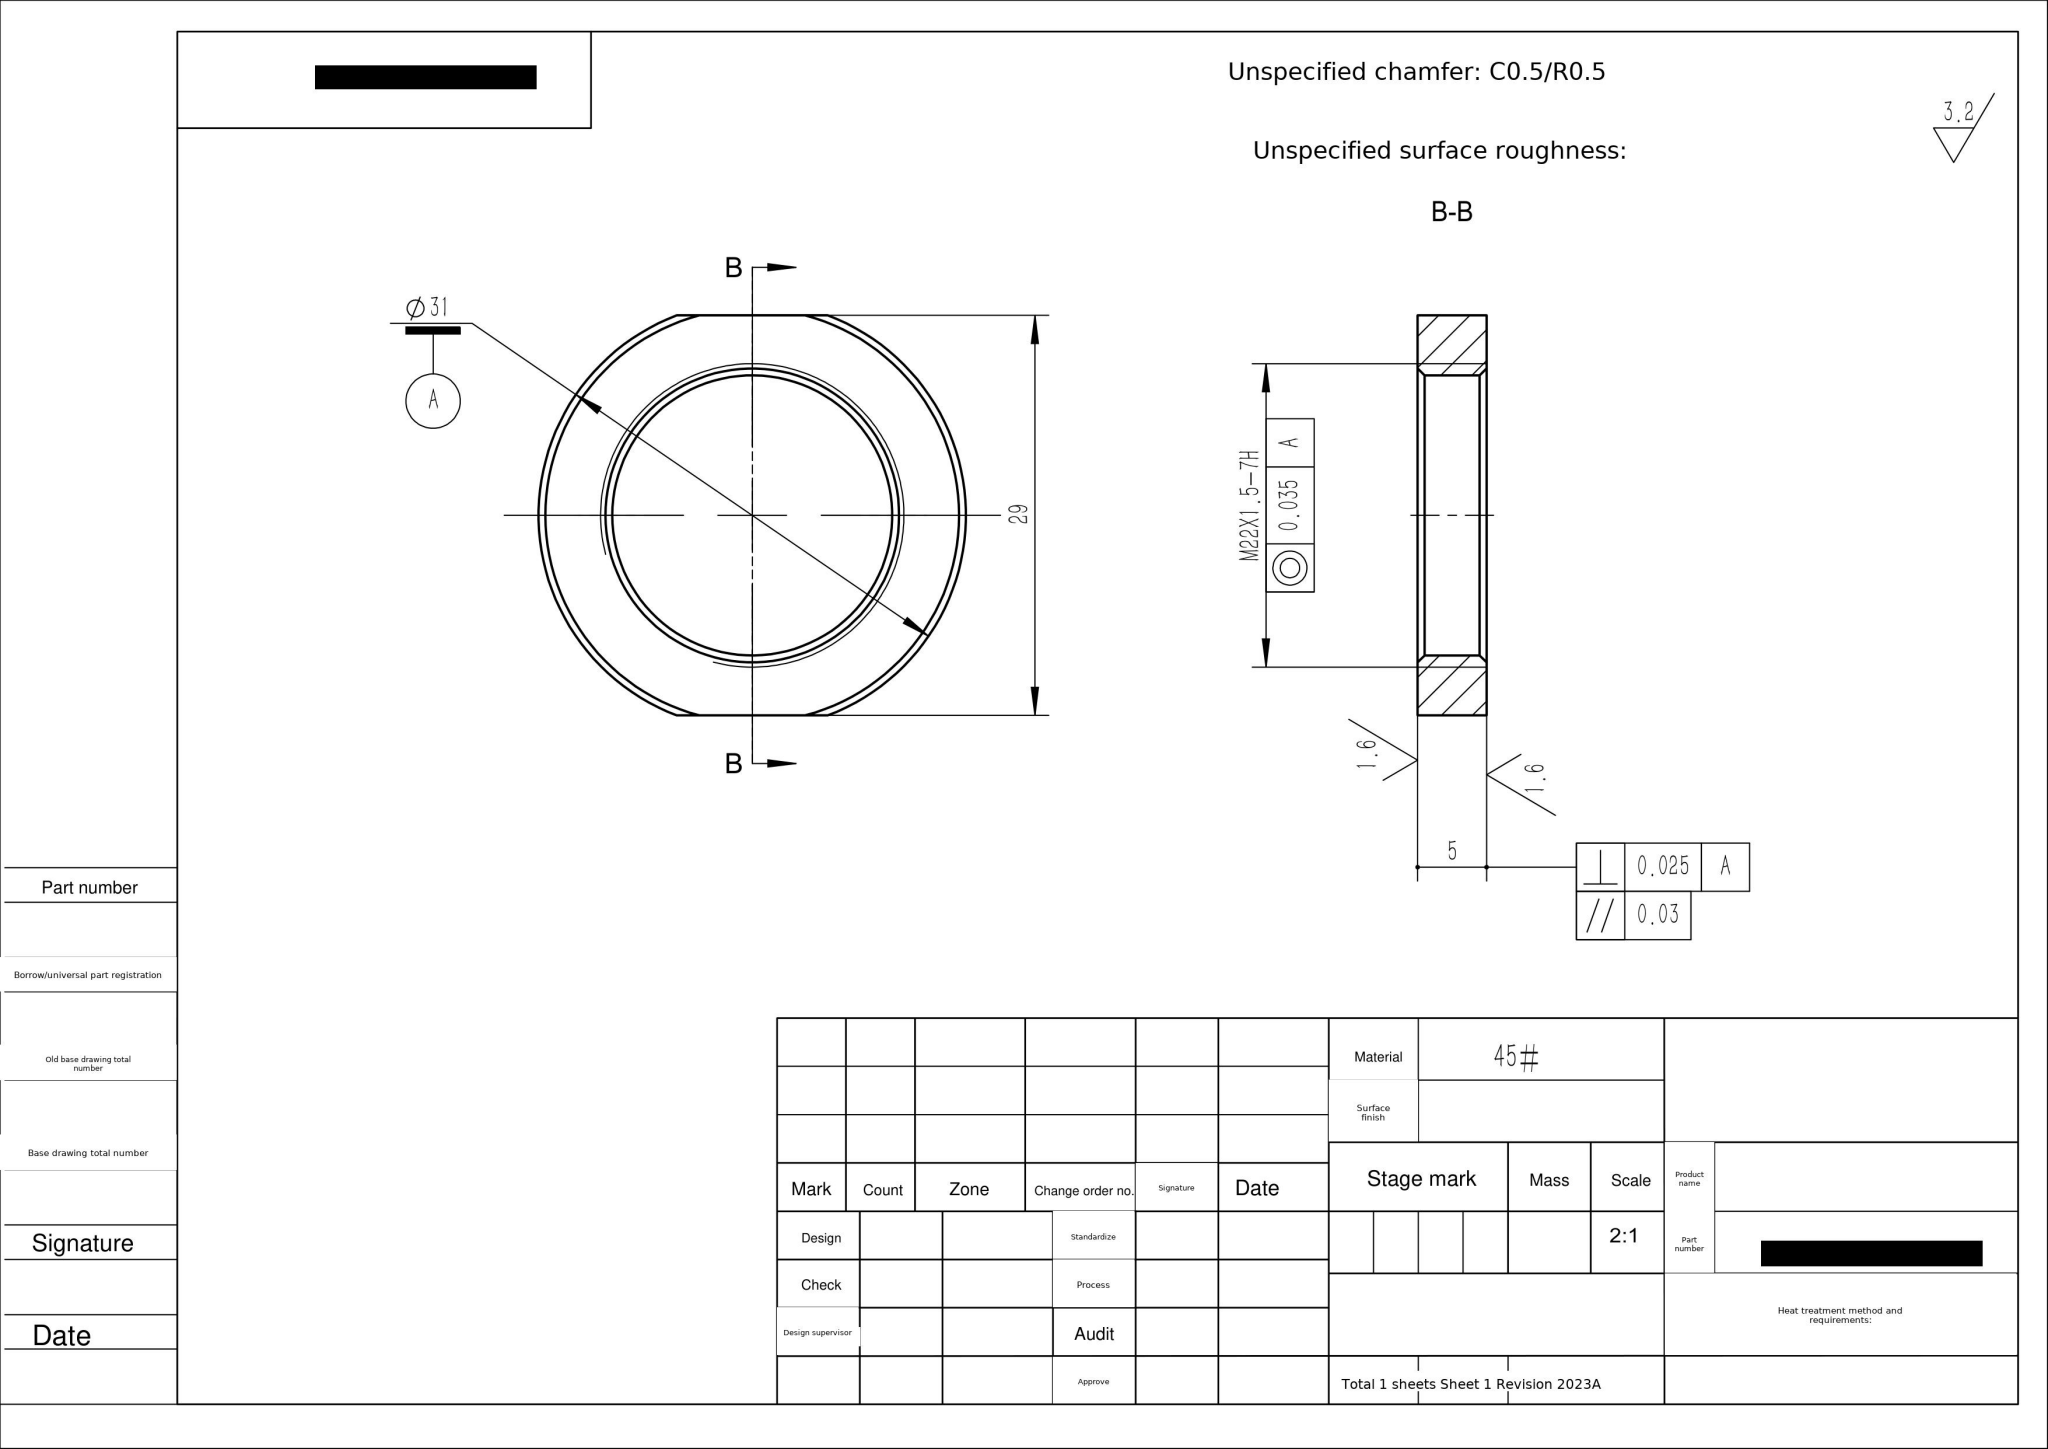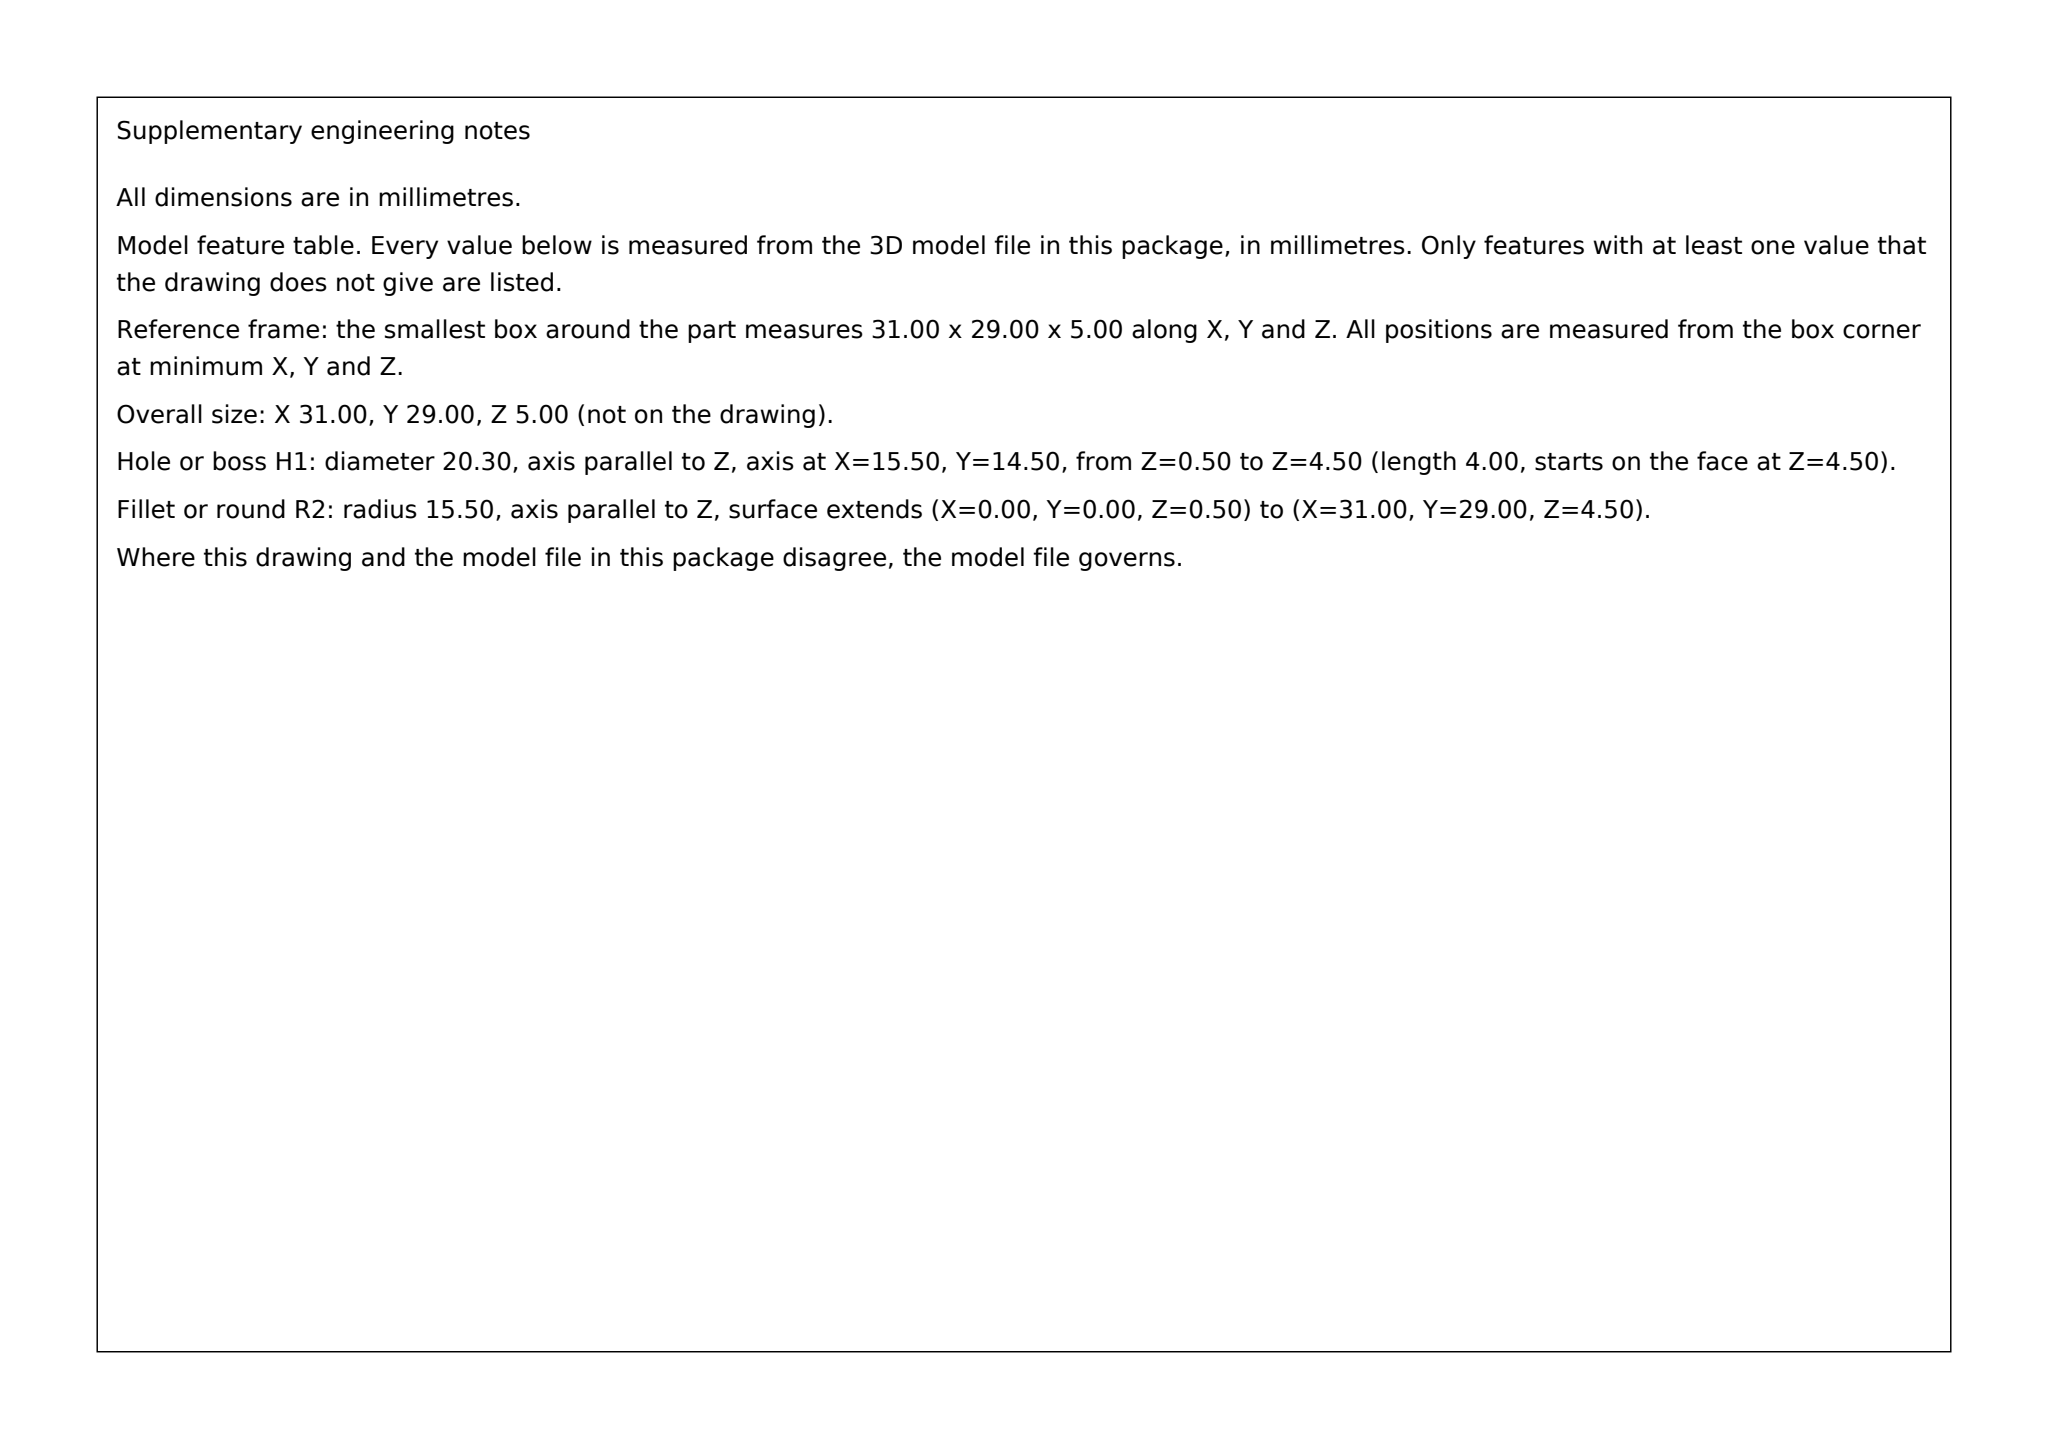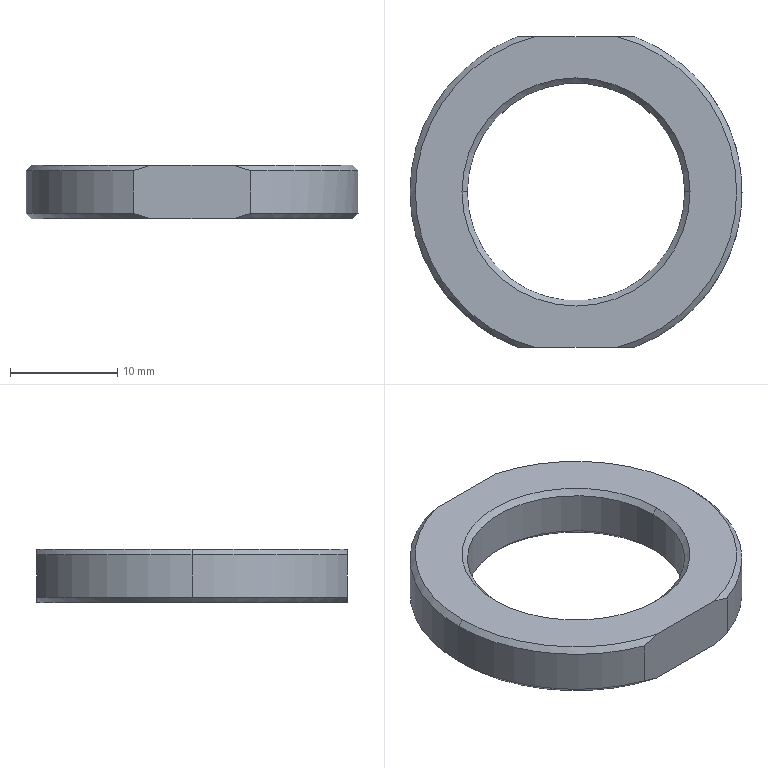Part | SolidWorks | mm | material 45# | 1 solid | 19 faces | box 31 x 29 x 5 mm | volume 2047 mm3 | cone 10 | cylinder 5 | plane 4 | commonest cylinder face diameters 31 x3 20.3 x2
build123d program:
from build123d import *

# Parameters (mm, degrees)
SKETCH1_R           = 15.5
SKETCH1_R_2         = 10.15
BOSS_EXTRUDE1_DEPTH = 5
CHAMFER1_SIZE       = 0.5
CHAMFER2_SIZE       = 0.5
SKETCH2_OUTSIDE_W   = 41.824
SKETCH2_OUTSIDE_H   = 41.824
SKETCH2_OUTSIDE_W_2 = 47.253
SKETCH2_OUTSIDE_H_2 = 29
CUT_EXTRUDE1_DEPTH  = 23.483


with BuildPart() as part:
    # Sketch1 → Boss-Extrude1 (new body)
    with BuildSketch(Plane.XY):
        Circle(SKETCH1_R)
        Circle(SKETCH1_R_2, mode=Mode.SUBTRACT)
    extrude(amount=BOSS_EXTRUDE1_DEPTH)

    # Chamfer1
    chamfer1_edges = [part.edges().sort_by_distance(p)[0] for p in [
        (-10.15, 0, 0),
        (-10.15, 0, 5),
    ]]
    chamfer(chamfer1_edges, length=CHAMFER1_SIZE)

    # Chamfer2
    chamfer2_edges = [part.edges().sort_by_distance(p)[0] for p in [
        (-15.5, 0, 0),
        (-15.5, 0, 5),
    ]]
    chamfer(chamfer2_edges, length=CHAMFER2_SIZE)

    # Sketch2 outside → Cut-Extrude1 (cut, through all)
    with BuildSketch(Plane.XY.offset(5)):
        Rectangle(SKETCH2_OUTSIDE_W, SKETCH2_OUTSIDE_H)
        Rectangle(SKETCH2_OUTSIDE_W_2, SKETCH2_OUTSIDE_H_2, mode=Mode.SUBTRACT)
    extrude(amount=-CUT_EXTRUDE1_DEPTH, mode=Mode.SUBTRACT)


solid = part.part
STEP:
#1=CARTESIAN_POINT('',(-10.15,0.,4.5));
#2=VERTEX_POINT('',#1);
#3=CARTESIAN_POINT('',(10.15,0.,4.5));
#4=VERTEX_POINT('',#3);
#5=CARTESIAN_POINT('',(0.,0.,4.5));
#6=DIRECTION('',(0.,0.,1.));
#7=DIRECTION('',(1.,0.,0.));
#8=AXIS2_PLACEMENT_3D('',#5,#6,#7);
#9=CIRCLE('',#8,10.15);
#10=EDGE_CURVE('',#2,#4,#9,.T.);
#11=ORIENTED_EDGE('',*,*,#10,.F.);
#12=CARTESIAN_POINT('',(-10.65,0.,5.));
#13=VERTEX_POINT('',#12);
#14=CARTESIAN_POINT('',(-10.15,0.,4.5));
#15=DIRECTION('',(-0.7071,0.,0.7071));
#16=VECTOR('',#15,1000.);
#17=LINE('',#14,#16);
#18=EDGE_CURVE('',#2,#13,#17,.T.);
#19=ORIENTED_EDGE('',*,*,#18,.T.);
#20=CARTESIAN_POINT('',(10.65,0.,5.));
#21=VERTEX_POINT('',#20);
#22=CARTESIAN_POINT('',(0.,0.,5.));
#23=DIRECTION('',(0.,0.,-1.));
#24=DIRECTION('',(1.,0.,0.));
#25=AXIS2_PLACEMENT_3D('',#22,#23,#24);
#26=CIRCLE('',#25,10.65);
#27=EDGE_CURVE('',#21,#13,#26,.T.);
#28=ORIENTED_EDGE('',*,*,#27,.F.);
#29=CARTESIAN_POINT('',(10.15,0.,4.5));
#30=DIRECTION('',(0.7071,0.,0.7071));
#31=VECTOR('',#30,1000.);
#32=LINE('',#29,#31);
#33=EDGE_CURVE('',#4,#21,#32,.T.);
#34=ORIENTED_EDGE('',*,*,#33,.F.);
#35=EDGE_LOOP('',(#11,#19,#28,#34));
#36=FACE_OUTER_BOUND('',#35,.T.);
#37=CARTESIAN_POINT('',(0.,0.,4.5));
#38=DIRECTION('',(0.,0.,1.));
#39=DIRECTION('',(1.,0.,0.));
#40=AXIS2_PLACEMENT_3D('',#37,#38,#39);
#41=CONICAL_SURFACE('',#40,10.15,0.7854);
#42=ADVANCED_FACE('',(#36),#41,.F.);
#43=CARTESIAN_POINT('',(10.15,0.,0.5));
#44=VERTEX_POINT('',#43);
#45=CARTESIAN_POINT('',(-10.15,0.,0.5));
#46=VERTEX_POINT('',#45);
#47=CARTESIAN_POINT('',(0.,0.,0.5));
#48=DIRECTION('',(0.,0.,-1.));
#49=DIRECTION('',(1.,0.,0.));
#50=AXIS2_PLACEMENT_3D('',#47,#48,#49);
#51=CIRCLE('',#50,10.15);
#52=EDGE_CURVE('',#44,#46,#51,.T.);
#53=ORIENTED_EDGE('',*,*,#52,.F.);
#54=CARTESIAN_POINT('',(10.65,0.,0.));
#55=VERTEX_POINT('',#54);
#56=CARTESIAN_POINT('',(10.65,0.,0.));
#57=DIRECTION('',(0.7071,0.,-0.7071));
#58=VECTOR('',#57,1000.);
#59=LINE('',#56,#58);
#60=EDGE_CURVE('',#44,#55,#59,.T.);
#61=ORIENTED_EDGE('',*,*,#60,.T.);
#62=CARTESIAN_POINT('',(-10.65,0.,0.));
#63=VERTEX_POINT('',#62);
#64=CARTESIAN_POINT('',(0.,0.,0.));
#65=DIRECTION('',(0.,0.,1.));
#66=DIRECTION('',(1.,0.,0.));
#67=AXIS2_PLACEMENT_3D('',#64,#65,#66);
#68=CIRCLE('',#67,10.65);
#69=EDGE_CURVE('',#63,#55,#68,.T.);
#70=ORIENTED_EDGE('',*,*,#69,.F.);
#71=CARTESIAN_POINT('',(-10.65,0.,0.));
#72=DIRECTION('',(-0.7071,0.,-0.7071));
#73=VECTOR('',#72,1000.);
#74=LINE('',#71,#73);
#75=EDGE_CURVE('',#46,#63,#74,.T.);
#76=ORIENTED_EDGE('',*,*,#75,.F.);
#77=EDGE_LOOP('',(#53,#61,#70,#76));
#78=FACE_OUTER_BOUND('',#77,.T.);
#79=CARTESIAN_POINT('',(0.,0.,0.));
#80=DIRECTION('',(0.,0.,-1.));
#81=DIRECTION('',(-1.,0.,0.));
#82=AXIS2_PLACEMENT_3D('',#79,#80,#81);
#83=CONICAL_SURFACE('',#82,10.65,0.7854);
#84=ADVANCED_FACE('',(#78),#83,.F.);
#85=ORIENTED_EDGE('',*,*,#10,.T.);
#86=CARTESIAN_POINT('',(10.15,0.,5.));
#87=DIRECTION('',(0.,0.,-1.));
#88=VECTOR('',#87,1000.);
#89=LINE('',#86,#88);
#90=EDGE_CURVE('',#4,#44,#89,.T.);
#91=ORIENTED_EDGE('',*,*,#90,.T.);
#92=ORIENTED_EDGE('',*,*,#52,.T.);
#93=CARTESIAN_POINT('',(-10.15,0.,5.));
#94=DIRECTION('',(0.,0.,-1.));
#95=VECTOR('',#94,1000.);
#96=LINE('',#93,#95);
#97=EDGE_CURVE('',#2,#46,#96,.T.);
#98=ORIENTED_EDGE('',*,*,#97,.F.);
#99=EDGE_LOOP('',(#85,#91,#92,#98));
#100=FACE_OUTER_BOUND('',#99,.T.);
#101=CARTESIAN_POINT('',(0.,0.,5.));
#102=DIRECTION('',(0.,0.,-1.));
#103=DIRECTION('',(-1.,0.,0.));
#104=AXIS2_PLACEMENT_3D('',#101,#102,#103);
#105=CYLINDRICAL_SURFACE('',#104,10.15);
#106=ADVANCED_FACE('',(#100),#105,.F.);
#107=CARTESIAN_POINT('',(-15.,0.,5.));
#108=VERTEX_POINT('',#107);
#109=CARTESIAN_POINT('',(-3.841,-14.5,5.));
#110=VERTEX_POINT('',#109);
#111=CARTESIAN_POINT('',(0.,0.,5.));
#112=DIRECTION('',(0.,0.,1.));
#113=DIRECTION('',(1.,0.,0.));
#114=AXIS2_PLACEMENT_3D('',#111,#112,#113);
#115=CIRCLE('',#114,15.);
#116=EDGE_CURVE('',#108,#110,#115,.T.);
#117=ORIENTED_EDGE('',*,*,#116,.F.);
#118=CARTESIAN_POINT('',(-15.5,0.,4.5));
#119=VERTEX_POINT('',#118);
#120=CARTESIAN_POINT('',(-15.,0.,5.));
#121=DIRECTION('',(-0.7071,0.,-0.7071));
#122=VECTOR('',#121,1000.);
#123=LINE('',#120,#122);
#124=EDGE_CURVE('',#108,#119,#123,.T.);
#125=ORIENTED_EDGE('',*,*,#124,.T.);
#126=CARTESIAN_POINT('',(-5.477,-14.5,4.5));
#127=VERTEX_POINT('',#126);
#128=CARTESIAN_POINT('',(0.,0.,4.5));
#129=DIRECTION('',(0.,0.,-1.));
#130=DIRECTION('',(1.,0.,0.));
#131=AXIS2_PLACEMENT_3D('',#128,#129,#130);
#132=CIRCLE('',#131,15.5);
#133=EDGE_CURVE('',#127,#119,#132,.T.);
#134=ORIENTED_EDGE('',*,*,#133,.F.);
#135=CARTESIAN_POINT('',(-5.477,-14.5,4.5));
#136=CARTESIAN_POINT('',(-4.941,-14.5,4.69));
#137=CARTESIAN_POINT('',(-4.396,-14.5,4.858));
#138=CARTESIAN_POINT('',(-3.841,-14.5,5.));
#139=B_SPLINE_CURVE_WITH_KNOTS('',3,(#135,#136,#137,#138),.UNSPECIFIED.,.F.,.F.,(4,4),(0.03164,0.03335),.UNSPECIFIED.);
#140=EDGE_CURVE('',#127,#110,#139,.T.);
#141=ORIENTED_EDGE('',*,*,#140,.T.);
#142=EDGE_LOOP('',(#117,#125,#134,#141));
#143=FACE_OUTER_BOUND('',#142,.T.);
#144=CARTESIAN_POINT('',(0.,0.,5.));
#145=DIRECTION('',(0.,0.,-1.));
#146=DIRECTION('',(-1.,0.,0.));
#147=AXIS2_PLACEMENT_3D('',#144,#145,#146);
#148=CONICAL_SURFACE('',#147,15.,0.7854);
#149=ADVANCED_FACE('',(#143),#148,.T.);
#150=CARTESIAN_POINT('',(15.,0.,0.));
#151=VERTEX_POINT('',#150);
#152=CARTESIAN_POINT('',(3.841,-14.5,0.));
#153=VERTEX_POINT('',#152);
#154=CARTESIAN_POINT('',(0.,0.,0.));
#155=DIRECTION('',(0.,0.,-1.));
#156=DIRECTION('',(1.,0.,0.));
#157=AXIS2_PLACEMENT_3D('',#154,#155,#156);
#158=CIRCLE('',#157,15.);
#159=EDGE_CURVE('',#151,#153,#158,.T.);
#160=ORIENTED_EDGE('',*,*,#159,.F.);
#161=CARTESIAN_POINT('',(15.5,0.,0.5));
#162=VERTEX_POINT('',#161);
#163=CARTESIAN_POINT('',(15.5,0.,0.5));
#164=DIRECTION('',(0.7071,0.,0.7071));
#165=VECTOR('',#164,1000.);
#166=LINE('',#163,#165);
#167=EDGE_CURVE('',#151,#162,#166,.T.);
#168=ORIENTED_EDGE('',*,*,#167,.T.);
#169=CARTESIAN_POINT('',(5.477,-14.5,0.5));
#170=VERTEX_POINT('',#169);
#171=CARTESIAN_POINT('',(0.,0.,0.5));
#172=DIRECTION('',(0.,0.,1.));
#173=DIRECTION('',(1.,0.,0.));
#174=AXIS2_PLACEMENT_3D('',#171,#172,#173);
#175=CIRCLE('',#174,15.5);
#176=EDGE_CURVE('',#170,#162,#175,.T.);
#177=ORIENTED_EDGE('',*,*,#176,.F.);
#178=CARTESIAN_POINT('',(5.477,-14.5,0.5));
#179=CARTESIAN_POINT('',(4.941,-14.5,0.3104));
#180=CARTESIAN_POINT('',(4.396,-14.5,0.1421));
#181=CARTESIAN_POINT('',(3.841,-14.5,0.));
#182=B_SPLINE_CURVE_WITH_KNOTS('',3,(#178,#179,#180,#181),.UNSPECIFIED.,.F.,.F.,(4,4),(0.03164,0.03335),.UNSPECIFIED.);
#183=EDGE_CURVE('',#170,#153,#182,.T.);
#184=ORIENTED_EDGE('',*,*,#183,.T.);
#185=EDGE_LOOP('',(#160,#168,#177,#184));
#186=FACE_OUTER_BOUND('',#185,.T.);
#187=CARTESIAN_POINT('',(0.,0.,0.5));
#188=DIRECTION('',(0.,0.,1.));
#189=DIRECTION('',(1.,0.,0.));
#190=AXIS2_PLACEMENT_3D('',#187,#188,#189);
#191=CONICAL_SURFACE('',#190,15.5,0.7854);
#192=ADVANCED_FACE('',(#186),#191,.T.);
#193=ORIENTED_EDGE('',*,*,#133,.T.);
#194=CARTESIAN_POINT('',(-15.5,0.,0.5));
#195=VERTEX_POINT('',#194);
#196=CARTESIAN_POINT('',(-15.5,0.,5.));
#197=DIRECTION('',(0.,0.,-1.));
#198=VECTOR('',#197,1000.);
#199=LINE('',#196,#198);
#200=EDGE_CURVE('',#119,#195,#199,.T.);
#201=ORIENTED_EDGE('',*,*,#200,.T.);
#202=CARTESIAN_POINT('',(-5.477,-14.5,0.5));
#203=VERTEX_POINT('',#202);
#204=CARTESIAN_POINT('',(0.,0.,0.5));
#205=DIRECTION('',(0.,0.,1.));
#206=DIRECTION('',(1.,0.,0.));
#207=AXIS2_PLACEMENT_3D('',#204,#205,#206);
#208=CIRCLE('',#207,15.5);
#209=EDGE_CURVE('',#195,#203,#208,.T.);
#210=ORIENTED_EDGE('',*,*,#209,.T.);
#211=CARTESIAN_POINT('',(-5.477,-14.5,5.));
#212=DIRECTION('',(0.,0.,-1.));
#213=VECTOR('',#212,1000.);
#214=LINE('',#211,#213);
#215=EDGE_CURVE('',#127,#203,#214,.T.);
#216=ORIENTED_EDGE('',*,*,#215,.F.);
#217=EDGE_LOOP('',(#193,#201,#210,#216));
#218=FACE_OUTER_BOUND('',#217,.T.);
#219=CARTESIAN_POINT('',(0.,0.,5.));
#220=DIRECTION('',(0.,0.,-1.));
#221=DIRECTION('',(-1.,0.,0.));
#222=AXIS2_PLACEMENT_3D('',#219,#220,#221);
#223=CYLINDRICAL_SURFACE('',#222,15.5);
#224=ADVANCED_FACE('',(#218),#223,.T.);
#225=ORIENTED_EDGE('',*,*,#27,.T.);
#226=CARTESIAN_POINT('',(0.,0.,5.));
#227=DIRECTION('',(0.,0.,-1.));
#228=DIRECTION('',(1.,0.,0.));
#229=AXIS2_PLACEMENT_3D('',#226,#227,#228);
#230=CIRCLE('',#229,10.65);
#231=EDGE_CURVE('',#13,#21,#230,.T.);
#232=ORIENTED_EDGE('',*,*,#231,.T.);
#233=EDGE_LOOP('',(#225,#232));
#234=FACE_BOUND('',#233,.T.);
#235=CARTESIAN_POINT('',(-3.841,14.5,5.));
#236=VERTEX_POINT('',#235);
#237=CARTESIAN_POINT('',(0.,0.,5.));
#238=DIRECTION('',(0.,0.,1.));
#239=DIRECTION('',(1.,0.,0.));
#240=AXIS2_PLACEMENT_3D('',#237,#238,#239);
#241=CIRCLE('',#240,15.);
#242=EDGE_CURVE('',#236,#108,#241,.T.);
#243=ORIENTED_EDGE('',*,*,#242,.T.);
#244=ORIENTED_EDGE('',*,*,#116,.T.);
#245=CARTESIAN_POINT('',(3.841,-14.5,5.));
#246=VERTEX_POINT('',#245);
#247=CARTESIAN_POINT('',(-23.626,-14.5,5.));
#248=DIRECTION('',(1.,0.,0.));
#249=VECTOR('',#248,1000.);
#250=LINE('',#247,#249);
#251=EDGE_CURVE('',#110,#246,#250,.T.);
#252=ORIENTED_EDGE('',*,*,#251,.T.);
#253=CARTESIAN_POINT('',(3.841,14.5,5.));
#254=VERTEX_POINT('',#253);
#255=CARTESIAN_POINT('',(0.,0.,5.));
#256=DIRECTION('',(0.,0.,1.));
#257=DIRECTION('',(1.,0.,0.));
#258=AXIS2_PLACEMENT_3D('',#255,#256,#257);
#259=CIRCLE('',#258,15.);
#260=EDGE_CURVE('',#246,#254,#259,.T.);
#261=ORIENTED_EDGE('',*,*,#260,.T.);
#262=CARTESIAN_POINT('',(-23.626,14.5,5.));
#263=DIRECTION('',(-1.,0.,0.));
#264=VECTOR('',#263,1000.);
#265=LINE('',#262,#264);
#266=EDGE_CURVE('',#254,#236,#265,.T.);
#267=ORIENTED_EDGE('',*,*,#266,.T.);
#268=EDGE_LOOP('',(#243,#244,#252,#261,#267));
#269=FACE_OUTER_BOUND('',#268,.T.);
#270=CARTESIAN_POINT('',(0.,0.,5.));
#271=DIRECTION('',(0.,0.,1.));
#272=DIRECTION('',(1.,0.,0.));
#273=AXIS2_PLACEMENT_3D('',#270,#271,#272);
#274=PLANE('',#273);
#275=ADVANCED_FACE('',(#234,#269),#274,.T.);
#276=ORIENTED_EDGE('',*,*,#69,.T.);
#277=CARTESIAN_POINT('',(0.,0.,0.));
#278=DIRECTION('',(0.,0.,1.));
#279=DIRECTION('',(1.,0.,0.));
#280=AXIS2_PLACEMENT_3D('',#277,#278,#279);
#281=CIRCLE('',#280,10.65);
#282=EDGE_CURVE('',#55,#63,#281,.T.);
#283=ORIENTED_EDGE('',*,*,#282,.T.);
#284=EDGE_LOOP('',(#276,#283));
#285=FACE_BOUND('',#284,.T.);
#286=CARTESIAN_POINT('',(-3.841,-14.5,0.));
#287=VERTEX_POINT('',#286);
#288=CARTESIAN_POINT('',(-23.626,-14.5,0.));
#289=DIRECTION('',(1.,0.,0.));
#290=VECTOR('',#289,1000.);
#291=LINE('',#288,#290);
#292=EDGE_CURVE('',#287,#153,#291,.T.);
#293=ORIENTED_EDGE('',*,*,#292,.F.);
#294=CARTESIAN_POINT('',(-3.841,14.5,0.));
#295=VERTEX_POINT('',#294);
#296=CARTESIAN_POINT('',(0.,0.,0.));
#297=DIRECTION('',(0.,0.,-1.));
#298=DIRECTION('',(1.,0.,0.));
#299=AXIS2_PLACEMENT_3D('',#296,#297,#298);
#300=CIRCLE('',#299,15.);
#301=EDGE_CURVE('',#287,#295,#300,.T.);
#302=ORIENTED_EDGE('',*,*,#301,.T.);
#303=CARTESIAN_POINT('',(3.841,14.5,0.));
#304=VERTEX_POINT('',#303);
#305=CARTESIAN_POINT('',(-23.626,14.5,0.));
#306=DIRECTION('',(-1.,0.,0.));
#307=VECTOR('',#306,1000.);
#308=LINE('',#305,#307);
#309=EDGE_CURVE('',#304,#295,#308,.T.);
#310=ORIENTED_EDGE('',*,*,#309,.F.);
#311=CARTESIAN_POINT('',(0.,0.,0.));
#312=DIRECTION('',(0.,0.,-1.));
#313=DIRECTION('',(1.,-0.,0.));
#314=AXIS2_PLACEMENT_3D('',#311,#312,#313);
#315=CIRCLE('',#314,15.);
#316=EDGE_CURVE('',#304,#151,#315,.T.);
#317=ORIENTED_EDGE('',*,*,#316,.T.);
#318=ORIENTED_EDGE('',*,*,#159,.T.);
#319=EDGE_LOOP('',(#293,#302,#310,#317,#318));
#320=FACE_OUTER_BOUND('',#319,.T.);
#321=CARTESIAN_POINT('',(0.,0.,0.));
#322=DIRECTION('',(0.,0.,1.));
#323=DIRECTION('',(1.,0.,0.));
#324=AXIS2_PLACEMENT_3D('',#321,#322,#323);
#325=PLANE('',#324);
#326=ADVANCED_FACE('',(#285,#320),#325,.F.);
#327=ORIENTED_EDGE('',*,*,#200,.F.);
#328=CARTESIAN_POINT('',(-5.477,14.5,4.5));
#329=VERTEX_POINT('',#328);
#330=CARTESIAN_POINT('',(0.,0.,4.5));
#331=DIRECTION('',(0.,0.,-1.));
#332=DIRECTION('',(1.,-0.,0.));
#333=AXIS2_PLACEMENT_3D('',#330,#331,#332);
#334=CIRCLE('',#333,15.5);
#335=EDGE_CURVE('',#119,#329,#334,.T.);
#336=ORIENTED_EDGE('',*,*,#335,.T.);
#337=CARTESIAN_POINT('',(-5.477,14.5,0.5));
#338=VERTEX_POINT('',#337);
#339=CARTESIAN_POINT('',(-5.477,14.5,5.));
#340=DIRECTION('',(0.,0.,1.));
#341=VECTOR('',#340,1000.);
#342=LINE('',#339,#341);
#343=EDGE_CURVE('',#338,#329,#342,.T.);
#344=ORIENTED_EDGE('',*,*,#343,.F.);
#345=CARTESIAN_POINT('',(0.,0.,0.5));
#346=DIRECTION('',(0.,0.,1.));
#347=DIRECTION('',(1.,0.,0.));
#348=AXIS2_PLACEMENT_3D('',#345,#346,#347);
#349=CIRCLE('',#348,15.5);
#350=EDGE_CURVE('',#338,#195,#349,.T.);
#351=ORIENTED_EDGE('',*,*,#350,.T.);
#352=EDGE_LOOP('',(#327,#336,#344,#351));
#353=FACE_OUTER_BOUND('',#352,.T.);
#354=CARTESIAN_POINT('',(0.,0.,5.));
#355=DIRECTION('',(0.,0.,-1.));
#356=DIRECTION('',(-1.,0.,0.));
#357=AXIS2_PLACEMENT_3D('',#354,#355,#356);
#358=CYLINDRICAL_SURFACE('',#357,15.5);
#359=ADVANCED_FACE('',(#353),#358,.T.);
#360=CARTESIAN_POINT('',(5.477,-14.5,4.5));
#361=VERTEX_POINT('',#360);
#362=CARTESIAN_POINT('',(5.477,-14.5,5.));
#363=DIRECTION('',(0.,0.,1.));
#364=VECTOR('',#363,1000.);
#365=LINE('',#362,#364);
#366=EDGE_CURVE('',#170,#361,#365,.T.);
#367=ORIENTED_EDGE('',*,*,#366,.F.);
#368=ORIENTED_EDGE('',*,*,#176,.T.);
#369=CARTESIAN_POINT('',(5.477,14.5,0.5));
#370=VERTEX_POINT('',#369);
#371=CARTESIAN_POINT('',(0.,0.,0.5));
#372=DIRECTION('',(0.,0.,1.));
#373=DIRECTION('',(1.,0.,0.));
#374=AXIS2_PLACEMENT_3D('',#371,#372,#373);
#375=CIRCLE('',#374,15.5);
#376=EDGE_CURVE('',#162,#370,#375,.T.);
#377=ORIENTED_EDGE('',*,*,#376,.T.);
#378=CARTESIAN_POINT('',(5.477,14.5,4.5));
#379=VERTEX_POINT('',#378);
#380=CARTESIAN_POINT('',(5.477,14.5,5.));
#381=DIRECTION('',(0.,0.,-1.));
#382=VECTOR('',#381,1000.);
#383=LINE('',#380,#382);
#384=EDGE_CURVE('',#379,#370,#383,.T.);
#385=ORIENTED_EDGE('',*,*,#384,.F.);
#386=CARTESIAN_POINT('',(0.,0.,4.5));
#387=DIRECTION('',(0.,0.,-1.));
#388=DIRECTION('',(1.,0.,0.));
#389=AXIS2_PLACEMENT_3D('',#386,#387,#388);
#390=CIRCLE('',#389,15.5);
#391=EDGE_CURVE('',#379,#361,#390,.T.);
#392=ORIENTED_EDGE('',*,*,#391,.T.);
#393=EDGE_LOOP('',(#367,#368,#377,#385,#392));
#394=FACE_OUTER_BOUND('',#393,.T.);
#395=CARTESIAN_POINT('',(0.,0.,5.));
#396=DIRECTION('',(0.,0.,-1.));
#397=DIRECTION('',(-1.,0.,0.));
#398=AXIS2_PLACEMENT_3D('',#395,#396,#397);
#399=CYLINDRICAL_SURFACE('',#398,15.5);
#400=ADVANCED_FACE('',(#394),#399,.T.);
#401=ORIENTED_EDGE('',*,*,#167,.F.);
#402=ORIENTED_EDGE('',*,*,#316,.F.);
#403=CARTESIAN_POINT('',(3.841,14.5,0.));
#404=CARTESIAN_POINT('',(4.393,14.5,0.1414));
#405=CARTESIAN_POINT('',(4.938,14.5,0.3095));
#406=CARTESIAN_POINT('',(5.477,14.5,0.5));
#407=B_SPLINE_CURVE_WITH_KNOTS('',3,(#403,#404,#405,#406),.UNSPECIFIED.,.F.,.F.,(4,4),(0.04111,0.04282),.UNSPECIFIED.);
#408=EDGE_CURVE('',#304,#370,#407,.T.);
#409=ORIENTED_EDGE('',*,*,#408,.T.);
#410=ORIENTED_EDGE('',*,*,#376,.F.);
#411=EDGE_LOOP('',(#401,#402,#409,#410));
#412=FACE_OUTER_BOUND('',#411,.T.);
#413=CARTESIAN_POINT('',(0.,0.,0.5));
#414=DIRECTION('',(0.,0.,1.));
#415=DIRECTION('',(1.,0.,0.));
#416=AXIS2_PLACEMENT_3D('',#413,#414,#415);
#417=CONICAL_SURFACE('',#416,15.5,0.7854);
#418=ADVANCED_FACE('',(#412),#417,.T.);
#419=ORIENTED_EDGE('',*,*,#301,.F.);
#420=CARTESIAN_POINT('',(-3.841,-14.5,0.));
#421=CARTESIAN_POINT('',(-4.393,-14.5,0.1414));
#422=CARTESIAN_POINT('',(-4.938,-14.5,0.3095));
#423=CARTESIAN_POINT('',(-5.477,-14.5,0.5));
#424=B_SPLINE_CURVE_WITH_KNOTS('',3,(#420,#421,#422,#423),.UNSPECIFIED.,.F.,.F.,(4,4),(0.04111,0.04282),.UNSPECIFIED.);
#425=EDGE_CURVE('',#287,#203,#424,.T.);
#426=ORIENTED_EDGE('',*,*,#425,.T.);
#427=ORIENTED_EDGE('',*,*,#209,.F.);
#428=ORIENTED_EDGE('',*,*,#350,.F.);
#429=CARTESIAN_POINT('',(-5.477,14.5,0.5));
#430=CARTESIAN_POINT('',(-4.941,14.5,0.3104));
#431=CARTESIAN_POINT('',(-4.396,14.5,0.1421));
#432=CARTESIAN_POINT('',(-3.841,14.5,0.));
#433=B_SPLINE_CURVE_WITH_KNOTS('',3,(#429,#430,#431,#432),.UNSPECIFIED.,.F.,.F.,(4,4),(0.03164,0.03335),.UNSPECIFIED.);
#434=EDGE_CURVE('',#338,#295,#433,.T.);
#435=ORIENTED_EDGE('',*,*,#434,.T.);
#436=EDGE_LOOP('',(#419,#426,#427,#428,#435));
#437=FACE_OUTER_BOUND('',#436,.T.);
#438=CARTESIAN_POINT('',(0.,0.,0.5));
#439=DIRECTION('',(0.,0.,1.));
#440=DIRECTION('',(1.,0.,0.));
#441=AXIS2_PLACEMENT_3D('',#438,#439,#440);
#442=CONICAL_SURFACE('',#441,15.5,0.7854);
#443=ADVANCED_FACE('',(#437),#442,.T.);
#444=ORIENTED_EDGE('',*,*,#124,.F.);
#445=ORIENTED_EDGE('',*,*,#242,.F.);
#446=CARTESIAN_POINT('',(-3.841,14.5,5.));
#447=CARTESIAN_POINT('',(-4.393,14.5,4.859));
#448=CARTESIAN_POINT('',(-4.938,14.5,4.69));
#449=CARTESIAN_POINT('',(-5.477,14.5,4.5));
#450=B_SPLINE_CURVE_WITH_KNOTS('',3,(#446,#447,#448,#449),.UNSPECIFIED.,.F.,.F.,(4,4),(0.04111,0.04282),.UNSPECIFIED.);
#451=EDGE_CURVE('',#236,#329,#450,.T.);
#452=ORIENTED_EDGE('',*,*,#451,.T.);
#453=ORIENTED_EDGE('',*,*,#335,.F.);
#454=EDGE_LOOP('',(#444,#445,#452,#453));
#455=FACE_OUTER_BOUND('',#454,.T.);
#456=CARTESIAN_POINT('',(0.,0.,5.));
#457=DIRECTION('',(0.,0.,-1.));
#458=DIRECTION('',(-1.,0.,0.));
#459=AXIS2_PLACEMENT_3D('',#456,#457,#458);
#460=CONICAL_SURFACE('',#459,15.,0.7854);
#461=ADVANCED_FACE('',(#455),#460,.T.);
#462=ORIENTED_EDGE('',*,*,#260,.F.);
#463=CARTESIAN_POINT('',(3.841,-14.5,5.));
#464=CARTESIAN_POINT('',(4.393,-14.5,4.859));
#465=CARTESIAN_POINT('',(4.938,-14.5,4.69));
#466=CARTESIAN_POINT('',(5.477,-14.5,4.5));
#467=B_SPLINE_CURVE_WITH_KNOTS('',3,(#463,#464,#465,#466),.UNSPECIFIED.,.F.,.F.,(4,4),(0.04111,0.04282),.UNSPECIFIED.);
#468=EDGE_CURVE('',#246,#361,#467,.T.);
#469=ORIENTED_EDGE('',*,*,#468,.T.);
#470=ORIENTED_EDGE('',*,*,#391,.F.);
#471=CARTESIAN_POINT('',(5.477,14.5,4.5));
#472=CARTESIAN_POINT('',(4.941,14.5,4.69));
#473=CARTESIAN_POINT('',(4.396,14.5,4.858));
#474=CARTESIAN_POINT('',(3.841,14.5,5.));
#475=B_SPLINE_CURVE_WITH_KNOTS('',3,(#471,#472,#473,#474),.UNSPECIFIED.,.F.,.F.,(4,4),(0.03164,0.03335),.UNSPECIFIED.);
#476=EDGE_CURVE('',#379,#254,#475,.T.);
#477=ORIENTED_EDGE('',*,*,#476,.T.);
#478=EDGE_LOOP('',(#462,#469,#470,#477));
#479=FACE_OUTER_BOUND('',#478,.T.);
#480=CARTESIAN_POINT('',(0.,0.,5.));
#481=DIRECTION('',(0.,0.,-1.));
#482=DIRECTION('',(-1.,0.,0.));
#483=AXIS2_PLACEMENT_3D('',#480,#481,#482);
#484=CONICAL_SURFACE('',#483,15.,0.7854);
#485=ADVANCED_FACE('',(#479),#484,.T.);
#486=ORIENTED_EDGE('',*,*,#90,.F.);
#487=CARTESIAN_POINT('',(0.,0.,4.5));
#488=DIRECTION('',(0.,0.,1.));
#489=DIRECTION('',(1.,0.,0.));
#490=AXIS2_PLACEMENT_3D('',#487,#488,#489);
#491=CIRCLE('',#490,10.15);
#492=EDGE_CURVE('',#4,#2,#491,.T.);
#493=ORIENTED_EDGE('',*,*,#492,.T.);
#494=ORIENTED_EDGE('',*,*,#97,.T.);
#495=CARTESIAN_POINT('',(0.,0.,0.5));
#496=DIRECTION('',(0.,0.,-1.));
#497=DIRECTION('',(1.,0.,0.));
#498=AXIS2_PLACEMENT_3D('',#495,#496,#497);
#499=CIRCLE('',#498,10.15);
#500=EDGE_CURVE('',#46,#44,#499,.T.);
#501=ORIENTED_EDGE('',*,*,#500,.T.);
#502=EDGE_LOOP('',(#486,#493,#494,#501));
#503=FACE_OUTER_BOUND('',#502,.T.);
#504=CARTESIAN_POINT('',(0.,0.,5.));
#505=DIRECTION('',(0.,0.,-1.));
#506=DIRECTION('',(-1.,0.,0.));
#507=AXIS2_PLACEMENT_3D('',#504,#505,#506);
#508=CYLINDRICAL_SURFACE('',#507,10.15);
#509=ADVANCED_FACE('',(#503),#508,.F.);
#510=ORIENTED_EDGE('',*,*,#60,.F.);
#511=ORIENTED_EDGE('',*,*,#500,.F.);
#512=ORIENTED_EDGE('',*,*,#75,.T.);
#513=ORIENTED_EDGE('',*,*,#282,.F.);
#514=EDGE_LOOP('',(#510,#511,#512,#513));
#515=FACE_OUTER_BOUND('',#514,.T.);
#516=CARTESIAN_POINT('',(0.,0.,0.));
#517=DIRECTION('',(0.,0.,-1.));
#518=DIRECTION('',(-1.,0.,0.));
#519=AXIS2_PLACEMENT_3D('',#516,#517,#518);
#520=CONICAL_SURFACE('',#519,10.65,0.7854);
#521=ADVANCED_FACE('',(#515),#520,.F.);
#522=ORIENTED_EDGE('',*,*,#18,.F.);
#523=ORIENTED_EDGE('',*,*,#492,.F.);
#524=ORIENTED_EDGE('',*,*,#33,.T.);
#525=ORIENTED_EDGE('',*,*,#231,.F.);
#526=EDGE_LOOP('',(#522,#523,#524,#525));
#527=FACE_OUTER_BOUND('',#526,.T.);
#528=CARTESIAN_POINT('',(0.,0.,4.5));
#529=DIRECTION('',(0.,0.,1.));
#530=DIRECTION('',(1.,0.,0.));
#531=AXIS2_PLACEMENT_3D('',#528,#529,#530);
#532=CONICAL_SURFACE('',#531,10.15,0.7854);
#533=ADVANCED_FACE('',(#527),#532,.F.);
#534=ORIENTED_EDGE('',*,*,#309,.T.);
#535=ORIENTED_EDGE('',*,*,#434,.F.);
#536=ORIENTED_EDGE('',*,*,#343,.T.);
#537=ORIENTED_EDGE('',*,*,#451,.F.);
#538=ORIENTED_EDGE('',*,*,#266,.F.);
#539=ORIENTED_EDGE('',*,*,#476,.F.);
#540=ORIENTED_EDGE('',*,*,#384,.T.);
#541=ORIENTED_EDGE('',*,*,#408,.F.);
#542=EDGE_LOOP('',(#534,#535,#536,#537,#538,#539,#540,#541));
#543=FACE_OUTER_BOUND('',#542,.T.);
#544=CARTESIAN_POINT('',(-23.626,14.5,0.));
#545=DIRECTION('',(0.,1.,0.));
#546=DIRECTION('',(0.,0.,1.));
#547=AXIS2_PLACEMENT_3D('',#544,#545,#546);
#548=PLANE('',#547);
#549=ADVANCED_FACE('',(#543),#548,.T.);
#550=ORIENTED_EDGE('',*,*,#292,.T.);
#551=ORIENTED_EDGE('',*,*,#183,.F.);
#552=ORIENTED_EDGE('',*,*,#366,.T.);
#553=ORIENTED_EDGE('',*,*,#468,.F.);
#554=ORIENTED_EDGE('',*,*,#251,.F.);
#555=ORIENTED_EDGE('',*,*,#140,.F.);
#556=ORIENTED_EDGE('',*,*,#215,.T.);
#557=ORIENTED_EDGE('',*,*,#425,.F.);
#558=EDGE_LOOP('',(#550,#551,#552,#553,#554,#555,#556,#557));
#559=FACE_OUTER_BOUND('',#558,.T.);
#560=CARTESIAN_POINT('',(-23.626,-14.5,0.));
#561=DIRECTION('',(0.,-1.,0.));
#562=DIRECTION('',(0.,0.,-1.));
#563=AXIS2_PLACEMENT_3D('',#560,#561,#562);
#564=PLANE('',#563);
#565=ADVANCED_FACE('',(#559),#564,.T.);
#566=CLOSED_SHELL('',(#42,#84,#106,#149,#192,#224,#275,#326,#359,#400,#418,#443,#461,#485,#509,#521,#533,#549,#565));
#567=MANIFOLD_SOLID_BREP('',#566);
#568=CARTESIAN_POINT('',(0.,0.,0.));
#569=DIRECTION('',(0.,0.,1.));
#570=DIRECTION('',(1.,0.,0.));
#571=AXIS2_PLACEMENT_3D('',#568,#569,#570);
#572=(LENGTH_UNIT()NAMED_UNIT(*)SI_UNIT(.MILLI.,.METRE.));
#573=UNCERTAINTY_MEASURE_WITH_UNIT(LENGTH_MEASURE(0.00001),#572,'','');
#574=(NAMED_UNIT(*)PLANE_ANGLE_UNIT()SI_UNIT($,.RADIAN.));
#575=(NAMED_UNIT(*)SI_UNIT($,.STERADIAN.)SOLID_ANGLE_UNIT());
#576=(GEOMETRIC_REPRESENTATION_CONTEXT(3)GLOBAL_UNCERTAINTY_ASSIGNED_CONTEXT((#573))GLOBAL_UNIT_ASSIGNED_CONTEXT((#572,#574,#575))REPRESENTATION_CONTEXT('',''));
#577=ADVANCED_BREP_SHAPE_REPRESENTATION('',(#567,#571),#576);